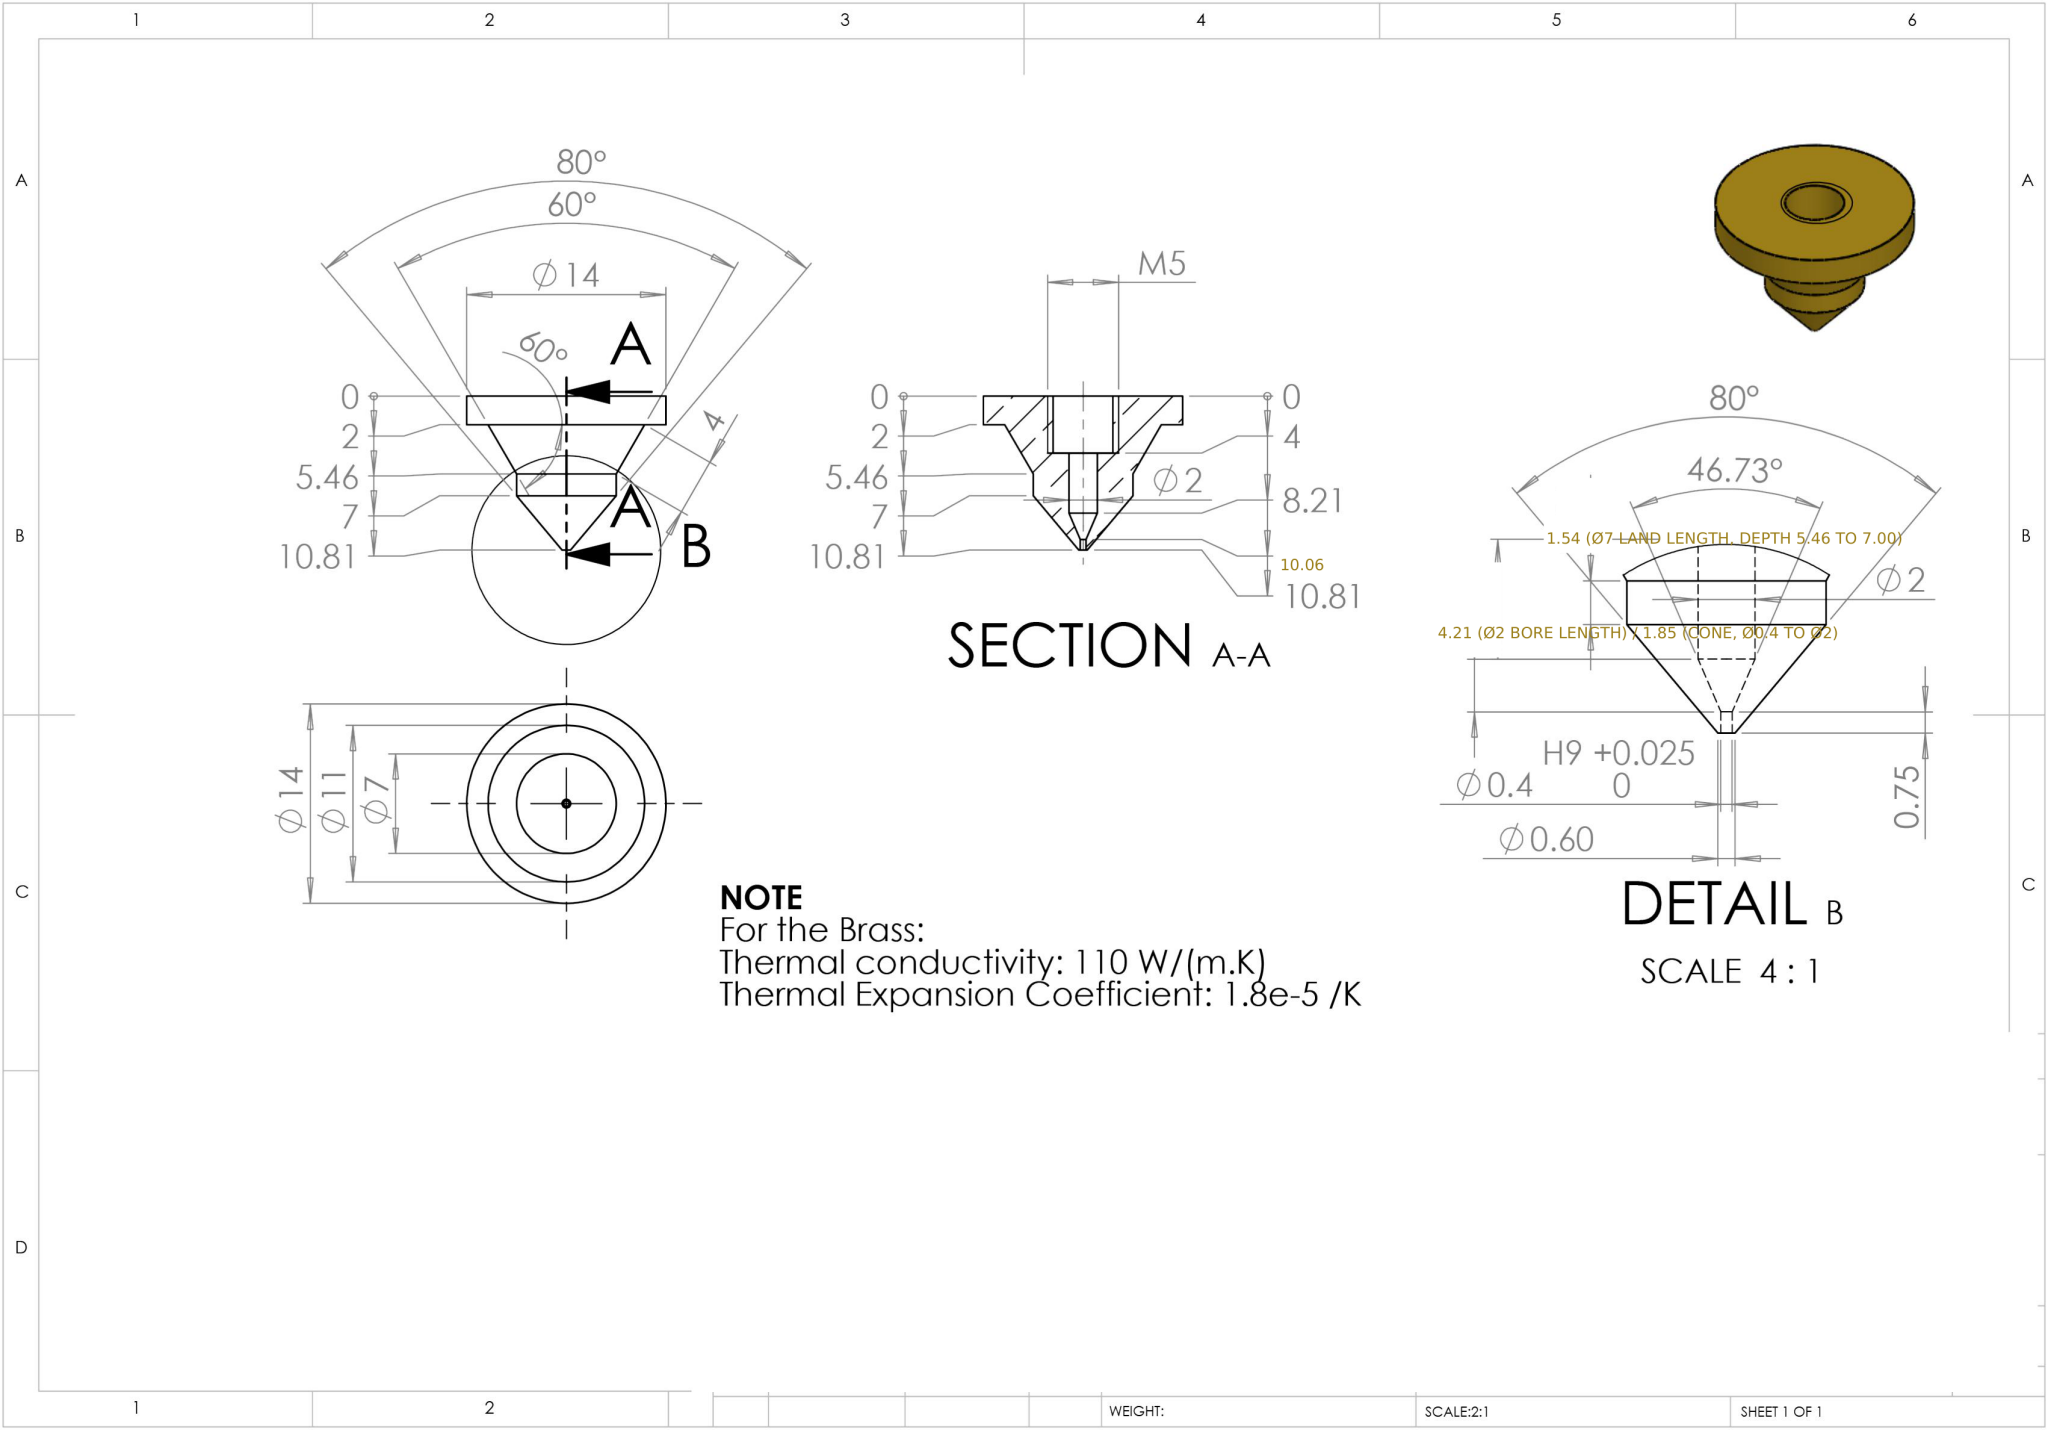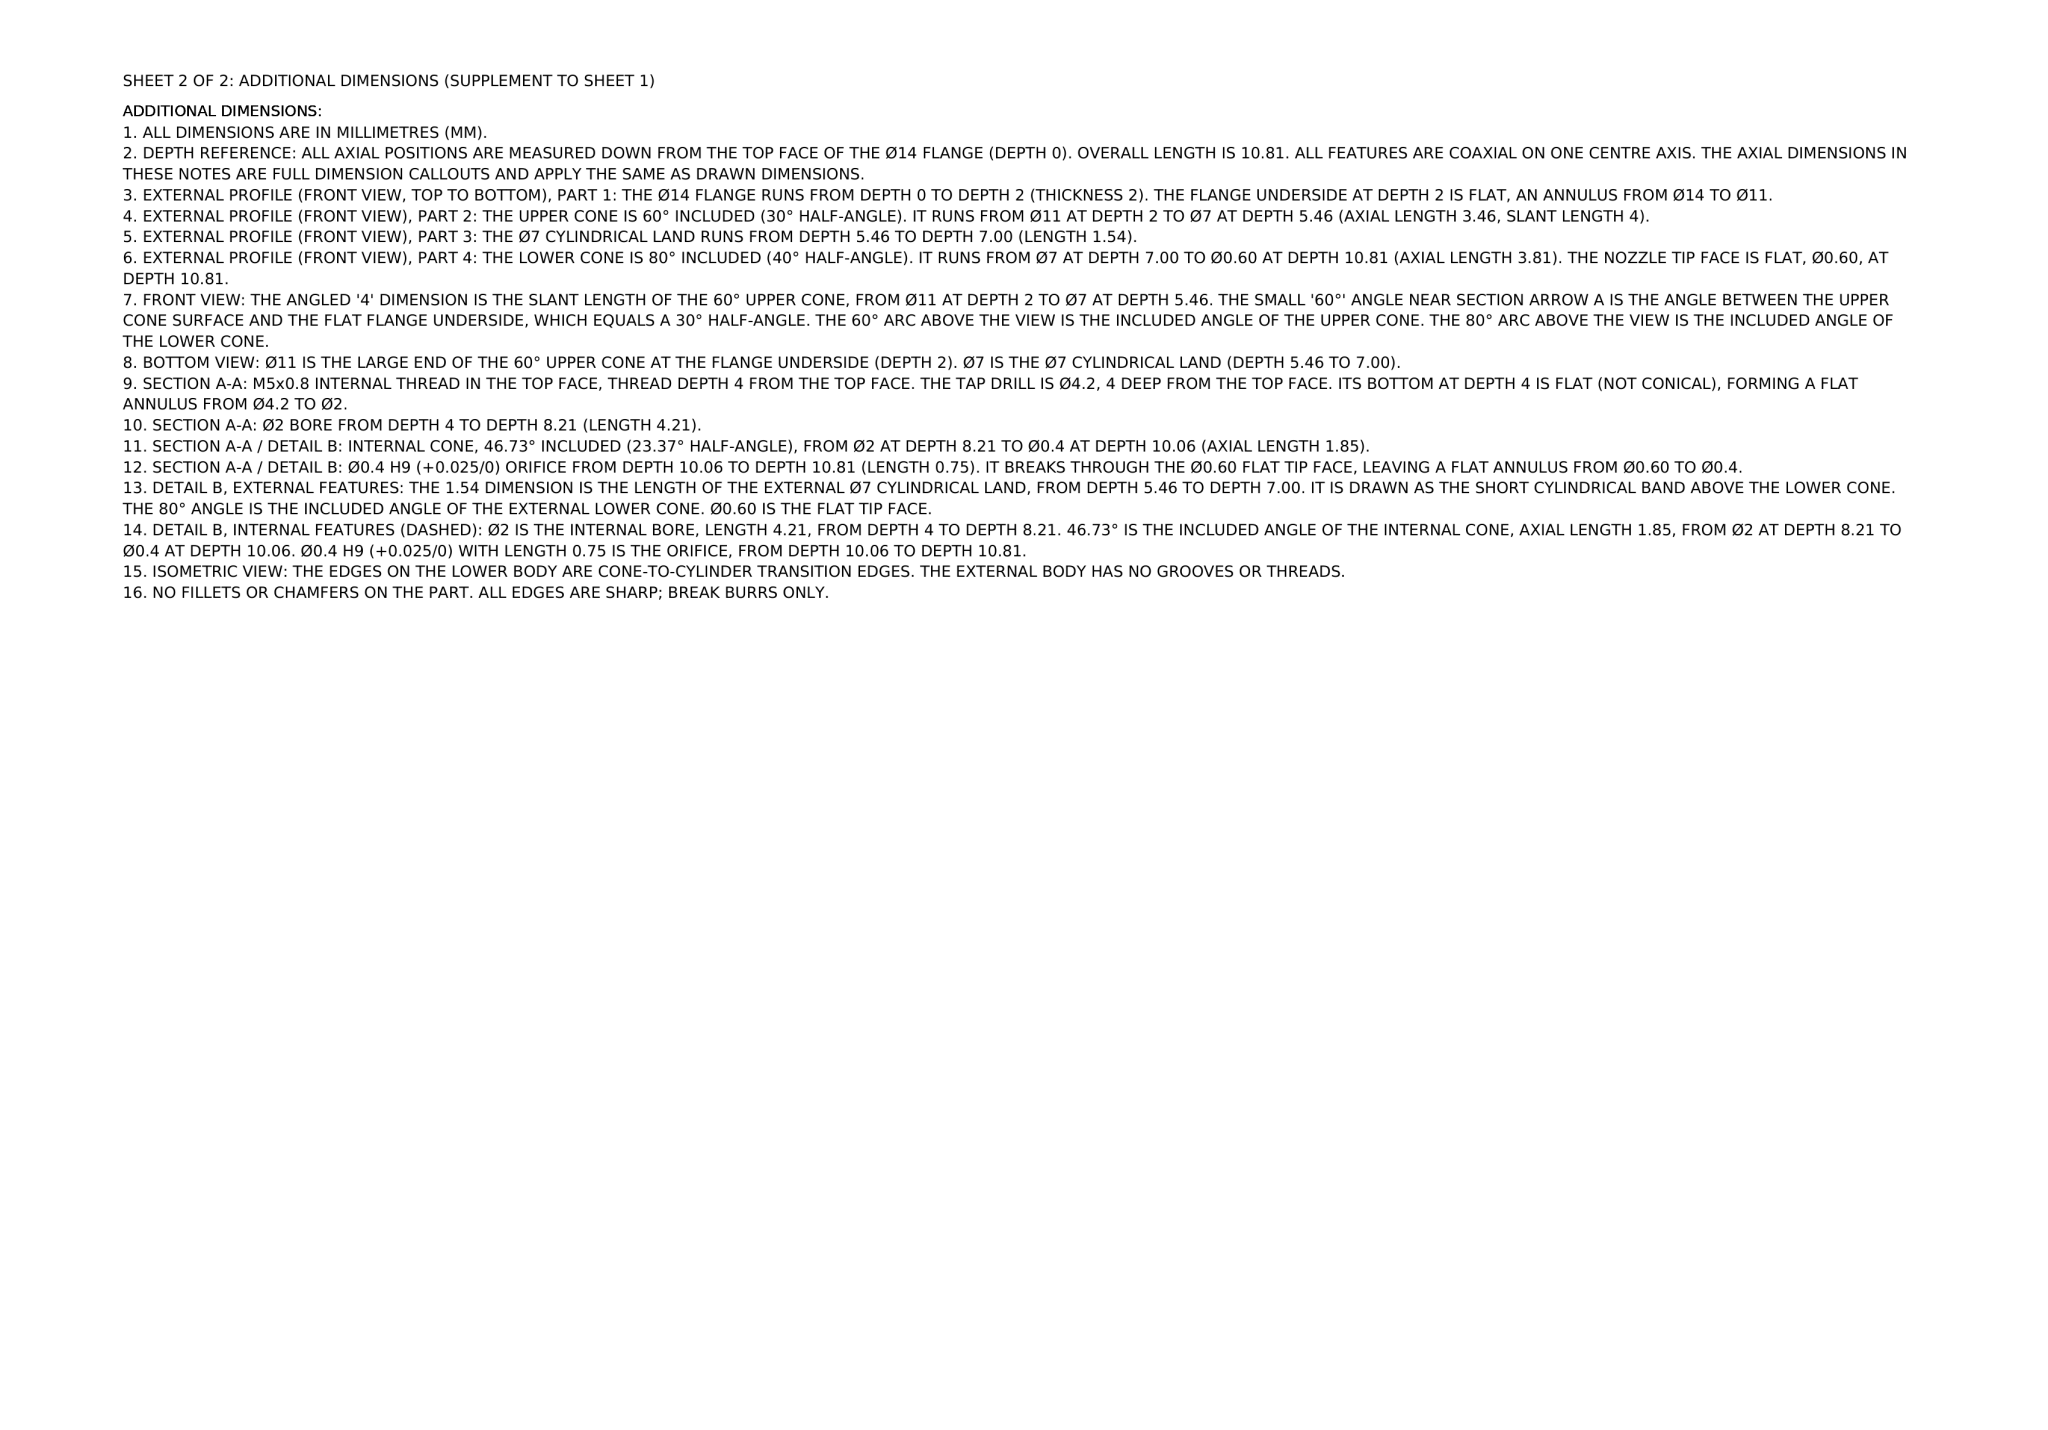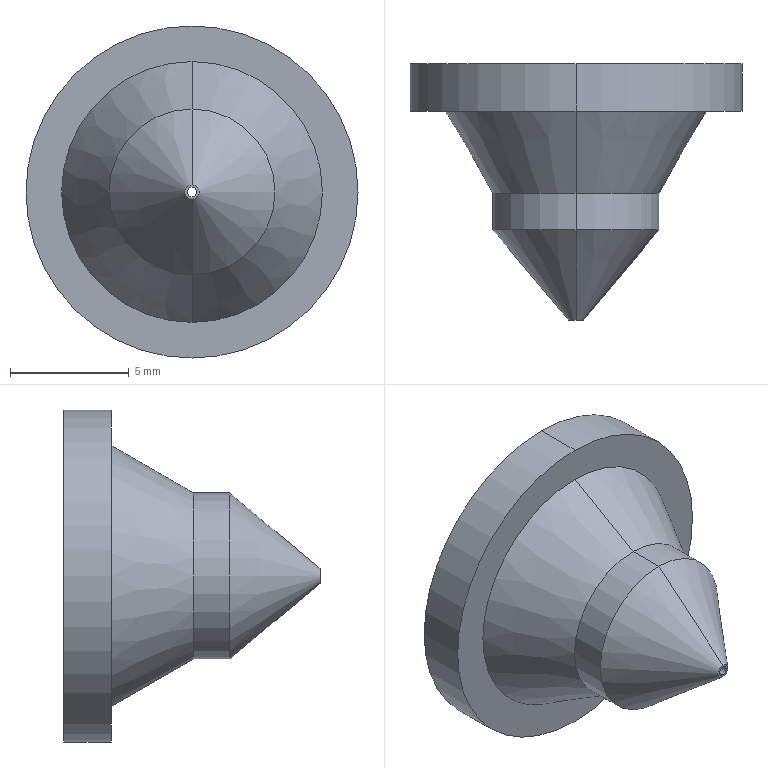Part | NX | mm | 1 solid | 20 faces | box 14 x 10.81 x 14 mm | volume 573 mm3 | cylinder 10 | cone 6 | plane 4 | commonest cylinder face diameters 4.2 x2 2 x2 14 x2 7 x2 0.4 x2
STEP:
#1=CARTESIAN_POINT('',(0.,5.35,-3.5));
#2=VERTEX_POINT('',#1);
#3=CARTESIAN_POINT('',(0.,5.35,3.5));
#4=VERTEX_POINT('',#3);
#5=CARTESIAN_POINT('',(0.,5.35,0.));
#6=DIRECTION('',(0.,-1.,0.));
#7=DIRECTION('',(0.,0.,-1.));
#8=AXIS2_PLACEMENT_3D('',#5,#6,#7);
#9=CIRCLE('',#8,3.5);
#10=EDGE_CURVE('',#2,#4,#9,.T.);
#11=ORIENTED_EDGE('',*,*,#10,.F.);
#12=CARTESIAN_POINT('',(0.,8.814,-5.5));
#13=VERTEX_POINT('',#12);
#14=CARTESIAN_POINT('',(0.,5.35,-3.5));
#15=DIRECTION('',(0.,0.866,-0.5));
#16=VECTOR('',#15,1000.);
#17=LINE('',#14,#16);
#18=EDGE_CURVE('',#2,#13,#17,.T.);
#19=ORIENTED_EDGE('',*,*,#18,.T.);
#20=CARTESIAN_POINT('',(0.,8.814,5.5));
#21=VERTEX_POINT('',#20);
#22=CARTESIAN_POINT('',(0.,8.814,0.));
#23=DIRECTION('',(0.,1.,0.));
#24=DIRECTION('',(0.,0.,-1.));
#25=AXIS2_PLACEMENT_3D('',#22,#23,#24);
#26=CIRCLE('',#25,5.5);
#27=EDGE_CURVE('',#21,#13,#26,.T.);
#28=ORIENTED_EDGE('',*,*,#27,.F.);
#29=CARTESIAN_POINT('',(0.,5.35,3.5));
#30=DIRECTION('',(0.,0.866,0.5));
#31=VECTOR('',#30,1000.);
#32=LINE('',#29,#31);
#33=EDGE_CURVE('',#4,#21,#32,.T.);
#34=ORIENTED_EDGE('',*,*,#33,.F.);
#35=EDGE_LOOP('',(#11,#19,#28,#34));
#36=FACE_OUTER_BOUND('',#35,.T.);
#37=CARTESIAN_POINT('',(0.,5.35,0.));
#38=DIRECTION('',(0.,1.,0.));
#39=DIRECTION('',(0.,0.,1.));
#40=AXIS2_PLACEMENT_3D('',#37,#38,#39);
#41=CONICAL_SURFACE('',#40,3.5,0.5236);
#42=ADVANCED_FACE('',(#36),#41,.T.);
#43=CARTESIAN_POINT('',(0.,6.814,-2.1));
#44=VERTEX_POINT('',#43);
#45=CARTESIAN_POINT('',(0.,6.814,2.1));
#46=VERTEX_POINT('',#45);
#47=CARTESIAN_POINT('',(0.,6.814,0.));
#48=DIRECTION('',(0.,1.,0.));
#49=DIRECTION('',(0.,0.,1.));
#50=AXIS2_PLACEMENT_3D('',#47,#48,#49);
#51=CIRCLE('',#50,2.1);
#52=EDGE_CURVE('',#44,#46,#51,.T.);
#53=ORIENTED_EDGE('',*,*,#52,.F.);
#54=CARTESIAN_POINT('',(0.,10.814,-2.1));
#55=VERTEX_POINT('',#54);
#56=CARTESIAN_POINT('',(0.,10.814,-2.1));
#57=DIRECTION('',(0.,1.,0.));
#58=VECTOR('',#57,1000.);
#59=LINE('',#56,#58);
#60=EDGE_CURVE('',#44,#55,#59,.T.);
#61=ORIENTED_EDGE('',*,*,#60,.T.);
#62=CARTESIAN_POINT('',(0.,10.814,2.1));
#63=VERTEX_POINT('',#62);
#64=CARTESIAN_POINT('',(0.,10.814,0.));
#65=DIRECTION('',(0.,1.,0.));
#66=DIRECTION('',(0.,0.,1.));
#67=AXIS2_PLACEMENT_3D('',#64,#65,#66);
#68=CIRCLE('',#67,2.1);
#69=EDGE_CURVE('',#55,#63,#68,.T.);
#70=ORIENTED_EDGE('',*,*,#69,.T.);
#71=CARTESIAN_POINT('',(0.,10.814,2.1));
#72=DIRECTION('',(0.,1.,0.));
#73=VECTOR('',#72,1000.);
#74=LINE('',#71,#73);
#75=EDGE_CURVE('',#46,#63,#74,.T.);
#76=ORIENTED_EDGE('',*,*,#75,.F.);
#77=EDGE_LOOP('',(#53,#61,#70,#76));
#78=FACE_OUTER_BOUND('',#77,.T.);
#79=CARTESIAN_POINT('',(0.,10.814,0.));
#80=DIRECTION('',(0.,1.,0.));
#81=DIRECTION('',(0.,0.,1.));
#82=AXIS2_PLACEMENT_3D('',#79,#80,#81);
#83=CYLINDRICAL_SURFACE('',#82,2.1);
#84=ADVANCED_FACE('',(#78),#83,.F.);
#85=CARTESIAN_POINT('',(0.,0.7484,0.2));
#86=VERTEX_POINT('',#85);
#87=CARTESIAN_POINT('',(0.,0.7484,-0.2));
#88=VERTEX_POINT('',#87);
#89=CARTESIAN_POINT('',(0.,0.7484,0.));
#90=DIRECTION('',(0.,-1.,0.));
#91=DIRECTION('',(0.,0.,-1.));
#92=AXIS2_PLACEMENT_3D('',#89,#90,#91);
#93=CIRCLE('',#92,0.2);
#94=EDGE_CURVE('',#86,#88,#93,.T.);
#95=ORIENTED_EDGE('',*,*,#94,.T.);
#96=CARTESIAN_POINT('',(0.,2.6,-1.));
#97=VERTEX_POINT('',#96);
#98=CARTESIAN_POINT('',(0.,2.6,-1.));
#99=DIRECTION('',(0.,0.918,-0.3966));
#100=VECTOR('',#99,1000.);
#101=LINE('',#98,#100);
#102=EDGE_CURVE('',#88,#97,#101,.T.);
#103=ORIENTED_EDGE('',*,*,#102,.T.);
#104=CARTESIAN_POINT('',(0.,2.6,1.));
#105=VERTEX_POINT('',#104);
#106=CARTESIAN_POINT('',(0.,2.6,0.));
#107=DIRECTION('',(0.,-1.,0.));
#108=DIRECTION('',(0.,0.,-1.));
#109=AXIS2_PLACEMENT_3D('',#106,#107,#108);
#110=CIRCLE('',#109,1.);
#111=EDGE_CURVE('',#105,#97,#110,.T.);
#112=ORIENTED_EDGE('',*,*,#111,.F.);
#113=CARTESIAN_POINT('',(0.,2.6,1.));
#114=DIRECTION('',(0.,0.918,0.3966));
#115=VECTOR('',#114,1000.);
#116=LINE('',#113,#115);
#117=EDGE_CURVE('',#86,#105,#116,.T.);
#118=ORIENTED_EDGE('',*,*,#117,.F.);
#119=EDGE_LOOP('',(#95,#103,#112,#118));
#120=FACE_OUTER_BOUND('',#119,.T.);
#121=CARTESIAN_POINT('',(0.,2.6,0.));
#122=DIRECTION('',(0.,1.,0.));
#123=DIRECTION('',(0.,0.,1.));
#124=AXIS2_PLACEMENT_3D('',#121,#122,#123);
#125=CONICAL_SURFACE('',#124,1.,0.4078);
#126=ADVANCED_FACE('',(#120),#125,.F.);
#127=CARTESIAN_POINT('',(0.,6.814,-1.));
#128=VERTEX_POINT('',#127);
#129=CARTESIAN_POINT('',(0.,6.814,1.));
#130=VERTEX_POINT('',#129);
#131=CARTESIAN_POINT('',(0.,6.814,0.));
#132=DIRECTION('',(0.,1.,0.));
#133=DIRECTION('',(0.,0.,1.));
#134=AXIS2_PLACEMENT_3D('',#131,#132,#133);
#135=CIRCLE('',#134,1.);
#136=EDGE_CURVE('',#128,#130,#135,.T.);
#137=ORIENTED_EDGE('',*,*,#136,.T.);
#138=CARTESIAN_POINT('',(0.,0.,1.));
#139=DIRECTION('',(0.,-1.,0.));
#140=VECTOR('',#139,1000.);
#141=LINE('',#138,#140);
#142=EDGE_CURVE('',#130,#105,#141,.T.);
#143=ORIENTED_EDGE('',*,*,#142,.T.);
#144=ORIENTED_EDGE('',*,*,#111,.T.);
#145=CARTESIAN_POINT('',(0.,0.,-1.));
#146=DIRECTION('',(0.,-1.,0.));
#147=VECTOR('',#146,1000.);
#148=LINE('',#145,#147);
#149=EDGE_CURVE('',#128,#97,#148,.T.);
#150=ORIENTED_EDGE('',*,*,#149,.F.);
#151=EDGE_LOOP('',(#137,#143,#144,#150));
#152=FACE_OUTER_BOUND('',#151,.T.);
#153=CARTESIAN_POINT('',(0.,0.,0.));
#154=DIRECTION('',(0.,-1.,0.));
#155=DIRECTION('',(0.,0.,-1.));
#156=AXIS2_PLACEMENT_3D('',#153,#154,#155);
#157=CYLINDRICAL_SURFACE('',#156,1.);
#158=ADVANCED_FACE('',(#152),#157,.F.);
#159=CARTESIAN_POINT('',(0.,10.814,-7.));
#160=VERTEX_POINT('',#159);
#161=CARTESIAN_POINT('',(0.,10.814,7.));
#162=VERTEX_POINT('',#161);
#163=CARTESIAN_POINT('',(0.,10.814,0.));
#164=DIRECTION('',(0.,-1.,0.));
#165=DIRECTION('',(0.,0.,-1.));
#166=AXIS2_PLACEMENT_3D('',#163,#164,#165);
#167=CIRCLE('',#166,7.);
#168=EDGE_CURVE('',#160,#162,#167,.T.);
#169=ORIENTED_EDGE('',*,*,#168,.T.);
#170=CARTESIAN_POINT('',(0.,8.814,7.));
#171=VERTEX_POINT('',#170);
#172=CARTESIAN_POINT('',(0.,0.,7.));
#173=DIRECTION('',(0.,-1.,0.));
#174=VECTOR('',#173,1000.);
#175=LINE('',#172,#174);
#176=EDGE_CURVE('',#162,#171,#175,.T.);
#177=ORIENTED_EDGE('',*,*,#176,.T.);
#178=CARTESIAN_POINT('',(0.,8.814,-7.));
#179=VERTEX_POINT('',#178);
#180=CARTESIAN_POINT('',(0.,8.814,0.));
#181=DIRECTION('',(0.,-1.,0.));
#182=DIRECTION('',(0.,0.,-1.));
#183=AXIS2_PLACEMENT_3D('',#180,#181,#182);
#184=CIRCLE('',#183,7.);
#185=EDGE_CURVE('',#179,#171,#184,.T.);
#186=ORIENTED_EDGE('',*,*,#185,.F.);
#187=CARTESIAN_POINT('',(0.,0.,-7.));
#188=DIRECTION('',(0.,-1.,0.));
#189=VECTOR('',#188,1000.);
#190=LINE('',#187,#189);
#191=EDGE_CURVE('',#160,#179,#190,.T.);
#192=ORIENTED_EDGE('',*,*,#191,.F.);
#193=EDGE_LOOP('',(#169,#177,#186,#192));
#194=FACE_OUTER_BOUND('',#193,.T.);
#195=CARTESIAN_POINT('',(0.,0.,0.));
#196=DIRECTION('',(0.,-1.,0.));
#197=DIRECTION('',(0.,0.,-1.));
#198=AXIS2_PLACEMENT_3D('',#195,#196,#197);
#199=CYLINDRICAL_SURFACE('',#198,7.);
#200=ADVANCED_FACE('',(#194),#199,.T.);
#201=ORIENTED_EDGE('',*,*,#10,.T.);
#202=CARTESIAN_POINT('',(0.,3.814,3.5));
#203=VERTEX_POINT('',#202);
#204=CARTESIAN_POINT('',(0.,0.,3.5));
#205=DIRECTION('',(0.,-1.,0.));
#206=VECTOR('',#205,1000.);
#207=LINE('',#204,#206);
#208=EDGE_CURVE('',#4,#203,#207,.T.);
#209=ORIENTED_EDGE('',*,*,#208,.T.);
#210=CARTESIAN_POINT('',(0.,3.814,-3.5));
#211=VERTEX_POINT('',#210);
#212=CARTESIAN_POINT('',(0.,3.814,0.));
#213=DIRECTION('',(0.,-1.,0.));
#214=DIRECTION('',(0.,0.,-1.));
#215=AXIS2_PLACEMENT_3D('',#212,#213,#214);
#216=CIRCLE('',#215,3.5);
#217=EDGE_CURVE('',#211,#203,#216,.T.);
#218=ORIENTED_EDGE('',*,*,#217,.F.);
#219=CARTESIAN_POINT('',(0.,0.,-3.5));
#220=DIRECTION('',(0.,-1.,0.));
#221=VECTOR('',#220,1000.);
#222=LINE('',#219,#221);
#223=EDGE_CURVE('',#2,#211,#222,.T.);
#224=ORIENTED_EDGE('',*,*,#223,.F.);
#225=EDGE_LOOP('',(#201,#209,#218,#224));
#226=FACE_OUTER_BOUND('',#225,.T.);
#227=CARTESIAN_POINT('',(0.,0.,0.));
#228=DIRECTION('',(0.,-1.,0.));
#229=DIRECTION('',(0.,0.,-1.));
#230=AXIS2_PLACEMENT_3D('',#227,#228,#229);
#231=CYLINDRICAL_SURFACE('',#230,3.5);
#232=ADVANCED_FACE('',(#226),#231,.T.);
#233=CARTESIAN_POINT('',(0.,0.,-0.3));
#234=VERTEX_POINT('',#233);
#235=CARTESIAN_POINT('',(0.,0.,0.3));
#236=VERTEX_POINT('',#235);
#237=CARTESIAN_POINT('',(0.,0.,0.));
#238=DIRECTION('',(0.,-1.,0.));
#239=DIRECTION('',(0.,0.,-1.));
#240=AXIS2_PLACEMENT_3D('',#237,#238,#239);
#241=CIRCLE('',#240,0.3);
#242=EDGE_CURVE('',#234,#236,#241,.T.);
#243=ORIENTED_EDGE('',*,*,#242,.F.);
#244=CARTESIAN_POINT('',(0.,0.,-0.3));
#245=DIRECTION('',(0.,0.766,-0.6428));
#246=VECTOR('',#245,1000.);
#247=LINE('',#244,#246);
#248=EDGE_CURVE('',#234,#211,#247,.T.);
#249=ORIENTED_EDGE('',*,*,#248,.T.);
#250=ORIENTED_EDGE('',*,*,#217,.T.);
#251=CARTESIAN_POINT('',(0.,0.,0.3));
#252=DIRECTION('',(0.,0.766,0.6428));
#253=VECTOR('',#252,1000.);
#254=LINE('',#251,#253);
#255=EDGE_CURVE('',#236,#203,#254,.T.);
#256=ORIENTED_EDGE('',*,*,#255,.F.);
#257=EDGE_LOOP('',(#243,#249,#250,#256));
#258=FACE_OUTER_BOUND('',#257,.T.);
#259=CARTESIAN_POINT('',(0.,0.,0.));
#260=DIRECTION('',(0.,1.,0.));
#261=DIRECTION('',(0.,0.,1.));
#262=AXIS2_PLACEMENT_3D('',#259,#260,#261);
#263=CONICAL_SURFACE('',#262,0.3,0.6981);
#264=ADVANCED_FACE('',(#258),#263,.T.);
#265=ORIENTED_EDGE('',*,*,#94,.F.);
#266=CARTESIAN_POINT('',(0.,0.,0.2));
#267=VERTEX_POINT('',#266);
#268=CARTESIAN_POINT('',(0.,0.,0.2));
#269=DIRECTION('',(0.,-1.,0.));
#270=VECTOR('',#269,1000.);
#271=LINE('',#268,#270);
#272=EDGE_CURVE('',#86,#267,#271,.T.);
#273=ORIENTED_EDGE('',*,*,#272,.T.);
#274=CARTESIAN_POINT('',(0.,0.,-0.2));
#275=VERTEX_POINT('',#274);
#276=CARTESIAN_POINT('',(0.,0.,0.));
#277=DIRECTION('',(0.,-1.,0.));
#278=DIRECTION('',(0.,0.,-1.));
#279=AXIS2_PLACEMENT_3D('',#276,#277,#278);
#280=CIRCLE('',#279,0.2);
#281=EDGE_CURVE('',#267,#275,#280,.T.);
#282=ORIENTED_EDGE('',*,*,#281,.T.);
#283=CARTESIAN_POINT('',(0.,0.,-0.2));
#284=DIRECTION('',(0.,-1.,0.));
#285=VECTOR('',#284,1000.);
#286=LINE('',#283,#285);
#287=EDGE_CURVE('',#88,#275,#286,.T.);
#288=ORIENTED_EDGE('',*,*,#287,.F.);
#289=EDGE_LOOP('',(#265,#273,#282,#288));
#290=FACE_OUTER_BOUND('',#289,.T.);
#291=CARTESIAN_POINT('',(0.,0.,0.));
#292=DIRECTION('',(0.,-1.,0.));
#293=DIRECTION('',(0.,0.,-1.));
#294=AXIS2_PLACEMENT_3D('',#291,#292,#293);
#295=CYLINDRICAL_SURFACE('',#294,0.2);
#296=ADVANCED_FACE('',(#290),#295,.F.);
#297=ORIENTED_EDGE('',*,*,#272,.F.);
#298=CARTESIAN_POINT('',(0.,0.7484,0.));
#299=DIRECTION('',(0.,-1.,0.));
#300=DIRECTION('',(0.,0.,-1.));
#301=AXIS2_PLACEMENT_3D('',#298,#299,#300);
#302=CIRCLE('',#301,0.2);
#303=EDGE_CURVE('',#88,#86,#302,.T.);
#304=ORIENTED_EDGE('',*,*,#303,.F.);
#305=ORIENTED_EDGE('',*,*,#287,.T.);
#306=CARTESIAN_POINT('',(0.,0.,0.));
#307=DIRECTION('',(0.,-1.,0.));
#308=DIRECTION('',(0.,0.,-1.));
#309=AXIS2_PLACEMENT_3D('',#306,#307,#308);
#310=CIRCLE('',#309,0.2);
#311=EDGE_CURVE('',#275,#267,#310,.T.);
#312=ORIENTED_EDGE('',*,*,#311,.T.);
#313=EDGE_LOOP('',(#297,#304,#305,#312));
#314=FACE_OUTER_BOUND('',#313,.T.);
#315=CARTESIAN_POINT('',(0.,0.,0.));
#316=DIRECTION('',(0.,-1.,0.));
#317=DIRECTION('',(0.,0.,-1.));
#318=AXIS2_PLACEMENT_3D('',#315,#316,#317);
#319=CYLINDRICAL_SURFACE('',#318,0.2);
#320=ADVANCED_FACE('',(#314),#319,.F.);
#321=CARTESIAN_POINT('',(0.,0.,0.));
#322=DIRECTION('',(0.,-1.,0.));
#323=DIRECTION('',(0.,0.,-1.));
#324=AXIS2_PLACEMENT_3D('',#321,#322,#323);
#325=CIRCLE('',#324,0.3);
#326=EDGE_CURVE('',#236,#234,#325,.T.);
#327=ORIENTED_EDGE('',*,*,#326,.T.);
#328=ORIENTED_EDGE('',*,*,#242,.T.);
#329=EDGE_LOOP('',(#327,#328));
#330=FACE_OUTER_BOUND('',#329,.T.);
#331=ORIENTED_EDGE('',*,*,#311,.F.);
#332=ORIENTED_EDGE('',*,*,#281,.F.);
#333=EDGE_LOOP('',(#331,#332));
#334=FACE_BOUND('',#333,.T.);
#335=CARTESIAN_POINT('',(0.2,0.,0.));
#336=DIRECTION('',(0.,-1.,0.));
#337=DIRECTION('',(0.,0.,-1.));
#338=AXIS2_PLACEMENT_3D('',#335,#336,#337);
#339=PLANE('',#338);
#340=ADVANCED_FACE('',(#330,#334),#339,.T.);
#341=ORIENTED_EDGE('',*,*,#248,.F.);
#342=ORIENTED_EDGE('',*,*,#326,.F.);
#343=ORIENTED_EDGE('',*,*,#255,.T.);
#344=CARTESIAN_POINT('',(0.,3.814,0.));
#345=DIRECTION('',(0.,-1.,0.));
#346=DIRECTION('',(0.,0.,-1.));
#347=AXIS2_PLACEMENT_3D('',#344,#345,#346);
#348=CIRCLE('',#347,3.5);
#349=EDGE_CURVE('',#203,#211,#348,.T.);
#350=ORIENTED_EDGE('',*,*,#349,.T.);
#351=EDGE_LOOP('',(#341,#342,#343,#350));
#352=FACE_OUTER_BOUND('',#351,.T.);
#353=CARTESIAN_POINT('',(0.,0.,0.));
#354=DIRECTION('',(0.,1.,0.));
#355=DIRECTION('',(0.,0.,1.));
#356=AXIS2_PLACEMENT_3D('',#353,#354,#355);
#357=CONICAL_SURFACE('',#356,0.3,0.6981);
#358=ADVANCED_FACE('',(#352),#357,.T.);
#359=ORIENTED_EDGE('',*,*,#208,.F.);
#360=CARTESIAN_POINT('',(0.,5.35,0.));
#361=DIRECTION('',(0.,-1.,0.));
#362=DIRECTION('',(0.,0.,-1.));
#363=AXIS2_PLACEMENT_3D('',#360,#361,#362);
#364=CIRCLE('',#363,3.5);
#365=EDGE_CURVE('',#4,#2,#364,.T.);
#366=ORIENTED_EDGE('',*,*,#365,.T.);
#367=ORIENTED_EDGE('',*,*,#223,.T.);
#368=ORIENTED_EDGE('',*,*,#349,.F.);
#369=EDGE_LOOP('',(#359,#366,#367,#368));
#370=FACE_OUTER_BOUND('',#369,.T.);
#371=CARTESIAN_POINT('',(0.,0.,0.));
#372=DIRECTION('',(0.,-1.,0.));
#373=DIRECTION('',(0.,0.,-1.));
#374=AXIS2_PLACEMENT_3D('',#371,#372,#373);
#375=CYLINDRICAL_SURFACE('',#374,3.5);
#376=ADVANCED_FACE('',(#370),#375,.T.);
#377=ORIENTED_EDGE('',*,*,#27,.T.);
#378=CARTESIAN_POINT('',(0.,8.814,0.));
#379=DIRECTION('',(0.,1.,0.));
#380=DIRECTION('',(0.,0.,-1.));
#381=AXIS2_PLACEMENT_3D('',#378,#379,#380);
#382=CIRCLE('',#381,5.5);
#383=EDGE_CURVE('',#13,#21,#382,.T.);
#384=ORIENTED_EDGE('',*,*,#383,.T.);
#385=EDGE_LOOP('',(#377,#384));
#386=FACE_BOUND('',#385,.T.);
#387=ORIENTED_EDGE('',*,*,#185,.T.);
#388=CARTESIAN_POINT('',(0.,8.814,0.));
#389=DIRECTION('',(0.,-1.,0.));
#390=DIRECTION('',(0.,0.,-1.));
#391=AXIS2_PLACEMENT_3D('',#388,#389,#390);
#392=CIRCLE('',#391,7.);
#393=EDGE_CURVE('',#171,#179,#392,.T.);
#394=ORIENTED_EDGE('',*,*,#393,.T.);
#395=EDGE_LOOP('',(#387,#394));
#396=FACE_OUTER_BOUND('',#395,.T.);
#397=CARTESIAN_POINT('',(3.5,8.814,0.));
#398=DIRECTION('',(0.,-1.,0.));
#399=DIRECTION('',(0.,0.,-1.));
#400=AXIS2_PLACEMENT_3D('',#397,#398,#399);
#401=PLANE('',#400);
#402=ADVANCED_FACE('',(#386,#396),#401,.T.);
#403=ORIENTED_EDGE('',*,*,#176,.F.);
#404=CARTESIAN_POINT('',(0.,10.814,0.));
#405=DIRECTION('',(0.,-1.,0.));
#406=DIRECTION('',(0.,0.,-1.));
#407=AXIS2_PLACEMENT_3D('',#404,#405,#406);
#408=CIRCLE('',#407,7.);
#409=EDGE_CURVE('',#162,#160,#408,.T.);
#410=ORIENTED_EDGE('',*,*,#409,.T.);
#411=ORIENTED_EDGE('',*,*,#191,.T.);
#412=ORIENTED_EDGE('',*,*,#393,.F.);
#413=EDGE_LOOP('',(#403,#410,#411,#412));
#414=FACE_OUTER_BOUND('',#413,.T.);
#415=CARTESIAN_POINT('',(0.,0.,0.));
#416=DIRECTION('',(0.,-1.,0.));
#417=DIRECTION('',(0.,0.,-1.));
#418=AXIS2_PLACEMENT_3D('',#415,#416,#417);
#419=CYLINDRICAL_SURFACE('',#418,7.);
#420=ADVANCED_FACE('',(#414),#419,.T.);
#421=CARTESIAN_POINT('',(0.,10.814,0.));
#422=DIRECTION('',(0.,1.,0.));
#423=DIRECTION('',(0.,0.,1.));
#424=AXIS2_PLACEMENT_3D('',#421,#422,#423);
#425=CIRCLE('',#424,2.1);
#426=EDGE_CURVE('',#63,#55,#425,.T.);
#427=ORIENTED_EDGE('',*,*,#426,.F.);
#428=ORIENTED_EDGE('',*,*,#69,.F.);
#429=EDGE_LOOP('',(#427,#428));
#430=FACE_BOUND('',#429,.T.);
#431=ORIENTED_EDGE('',*,*,#168,.F.);
#432=ORIENTED_EDGE('',*,*,#409,.F.);
#433=EDGE_LOOP('',(#431,#432));
#434=FACE_OUTER_BOUND('',#433,.T.);
#435=CARTESIAN_POINT('',(2.5,10.814,0.));
#436=DIRECTION('',(0.,1.,0.));
#437=DIRECTION('',(0.,0.,1.));
#438=AXIS2_PLACEMENT_3D('',#435,#436,#437);
#439=PLANE('',#438);
#440=ADVANCED_FACE('',(#430,#434),#439,.T.);
#441=ORIENTED_EDGE('',*,*,#142,.F.);
#442=CARTESIAN_POINT('',(0.,6.814,0.));
#443=DIRECTION('',(0.,1.,0.));
#444=DIRECTION('',(0.,0.,1.));
#445=AXIS2_PLACEMENT_3D('',#442,#443,#444);
#446=CIRCLE('',#445,1.);
#447=EDGE_CURVE('',#130,#128,#446,.T.);
#448=ORIENTED_EDGE('',*,*,#447,.T.);
#449=ORIENTED_EDGE('',*,*,#149,.T.);
#450=CARTESIAN_POINT('',(0.,2.6,0.));
#451=DIRECTION('',(0.,-1.,0.));
#452=DIRECTION('',(0.,0.,-1.));
#453=AXIS2_PLACEMENT_3D('',#450,#451,#452);
#454=CIRCLE('',#453,1.);
#455=EDGE_CURVE('',#97,#105,#454,.T.);
#456=ORIENTED_EDGE('',*,*,#455,.T.);
#457=EDGE_LOOP('',(#441,#448,#449,#456));
#458=FACE_OUTER_BOUND('',#457,.T.);
#459=CARTESIAN_POINT('',(0.,0.,0.));
#460=DIRECTION('',(0.,-1.,0.));
#461=DIRECTION('',(0.,0.,-1.));
#462=AXIS2_PLACEMENT_3D('',#459,#460,#461);
#463=CYLINDRICAL_SURFACE('',#462,1.);
#464=ADVANCED_FACE('',(#458),#463,.F.);
#465=ORIENTED_EDGE('',*,*,#102,.F.);
#466=ORIENTED_EDGE('',*,*,#303,.T.);
#467=ORIENTED_EDGE('',*,*,#117,.T.);
#468=ORIENTED_EDGE('',*,*,#455,.F.);
#469=EDGE_LOOP('',(#465,#466,#467,#468));
#470=FACE_OUTER_BOUND('',#469,.T.);
#471=CARTESIAN_POINT('',(0.,2.6,0.));
#472=DIRECTION('',(0.,1.,0.));
#473=DIRECTION('',(0.,0.,1.));
#474=AXIS2_PLACEMENT_3D('',#471,#472,#473);
#475=CONICAL_SURFACE('',#474,1.,0.4078);
#476=ADVANCED_FACE('',(#470),#475,.F.);
#477=ORIENTED_EDGE('',*,*,#60,.F.);
#478=CARTESIAN_POINT('',(0.,6.814,0.));
#479=DIRECTION('',(0.,1.,0.));
#480=DIRECTION('',(0.,0.,1.));
#481=AXIS2_PLACEMENT_3D('',#478,#479,#480);
#482=CIRCLE('',#481,2.1);
#483=EDGE_CURVE('',#46,#44,#482,.T.);
#484=ORIENTED_EDGE('',*,*,#483,.F.);
#485=ORIENTED_EDGE('',*,*,#75,.T.);
#486=ORIENTED_EDGE('',*,*,#426,.T.);
#487=EDGE_LOOP('',(#477,#484,#485,#486));
#488=FACE_OUTER_BOUND('',#487,.T.);
#489=CARTESIAN_POINT('',(0.,10.814,0.));
#490=DIRECTION('',(0.,1.,0.));
#491=DIRECTION('',(0.,0.,1.));
#492=AXIS2_PLACEMENT_3D('',#489,#490,#491);
#493=CYLINDRICAL_SURFACE('',#492,2.1);
#494=ADVANCED_FACE('',(#488),#493,.F.);
#495=ORIENTED_EDGE('',*,*,#18,.F.);
#496=ORIENTED_EDGE('',*,*,#365,.F.);
#497=ORIENTED_EDGE('',*,*,#33,.T.);
#498=ORIENTED_EDGE('',*,*,#383,.F.);
#499=EDGE_LOOP('',(#495,#496,#497,#498));
#500=FACE_OUTER_BOUND('',#499,.T.);
#501=CARTESIAN_POINT('',(0.,5.35,0.));
#502=DIRECTION('',(0.,1.,0.));
#503=DIRECTION('',(0.,0.,1.));
#504=AXIS2_PLACEMENT_3D('',#501,#502,#503);
#505=CONICAL_SURFACE('',#504,3.5,0.5236);
#506=ADVANCED_FACE('',(#500),#505,.T.);
#507=ORIENTED_EDGE('',*,*,#136,.F.);
#508=ORIENTED_EDGE('',*,*,#447,.F.);
#509=EDGE_LOOP('',(#507,#508));
#510=FACE_BOUND('',#509,.T.);
#511=ORIENTED_EDGE('',*,*,#483,.T.);
#512=ORIENTED_EDGE('',*,*,#52,.T.);
#513=EDGE_LOOP('',(#511,#512));
#514=FACE_OUTER_BOUND('',#513,.T.);
#515=CARTESIAN_POINT('',(0.,6.814,0.));
#516=DIRECTION('',(0.,1.,0.));
#517=DIRECTION('',(0.,0.,1.));
#518=AXIS2_PLACEMENT_3D('',#515,#516,#517);
#519=PLANE('',#518);
#520=ADVANCED_FACE('',(#510,#514),#519,.T.);
#521=CLOSED_SHELL('',(#42,#84,#126,#158,#200,#232,#264,#296,#320,#340,#358,#376,#402,#420,#440,#464,#476,#494,#506,#520));
#522=MANIFOLD_SOLID_BREP('',#521);
#523=CARTESIAN_POINT('',(0.,0.,0.));
#524=DIRECTION('',(0.,0.,1.));
#525=DIRECTION('',(1.,0.,0.));
#526=AXIS2_PLACEMENT_3D('',#523,#524,#525);
#527=(LENGTH_UNIT()NAMED_UNIT(*)SI_UNIT(.MILLI.,.METRE.));
#528=UNCERTAINTY_MEASURE_WITH_UNIT(LENGTH_MEASURE(0.00001),#527,'','');
#529=(NAMED_UNIT(*)PLANE_ANGLE_UNIT()SI_UNIT($,.RADIAN.));
#530=(NAMED_UNIT(*)SI_UNIT($,.STERADIAN.)SOLID_ANGLE_UNIT());
#531=(GEOMETRIC_REPRESENTATION_CONTEXT(3)GLOBAL_UNCERTAINTY_ASSIGNED_CONTEXT((#528))GLOBAL_UNIT_ASSIGNED_CONTEXT((#527,#529,#530))REPRESENTATION_CONTEXT('',''));
#532=ADVANCED_BREP_SHAPE_REPRESENTATION('',(#522,#526),#531);